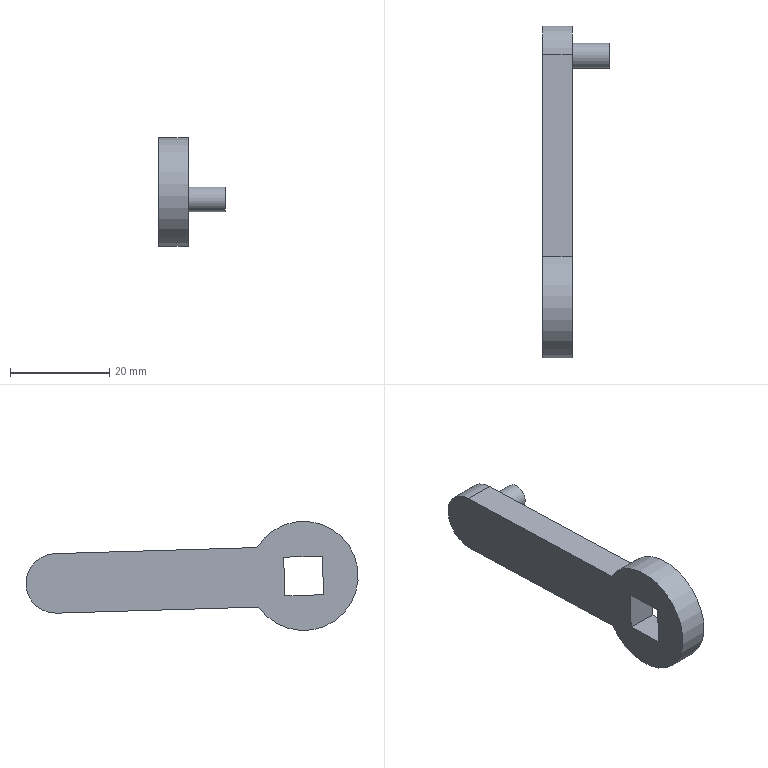Component | NX | ROCKER_CONNECTING_ROD | 1 solid | 12 faces | box 13.5 x 66.98 x 22 mm | volume 5252 mm3 | plane 9 | cylinder 3 | commonest cylinder face diameters 12 x1 22 x1 5 x1
STEP:
#1=CARTESIAN_POINT('',(0.,0.,0.));
#2=DIRECTION('',(0.,0.,1.));
#3=DIRECTION('',(1.,0.,0.));
#4=AXIS2_PLACEMENT_3D('',#1,#2,#3);
#5=CARTESIAN_POINT('',(35.,76.197,-15.982));
#6=VERTEX_POINT('',#5);
#7=CARTESIAN_POINT('',(35.,83.993,-16.221));
#8=VERTEX_POINT('',#7);
#9=CARTESIAN_POINT('',(35.,80.095,-16.101));
#10=DIRECTION('',(0.,0.9995,-0.03066));
#11=VECTOR('',#10,1.);
#12=LINE('',#9,#11);
#13=CARTESIAN_POINT('',(35.,129.953,-21.501));
#14=DIRECTION('',(1.,0.,0.));
#15=DIRECTION('',(0.,0.9995,-0.03004));
#16=AXIS2_PLACEMENT_3D('',#13,#14,#15);
#17=PLANE('',#16);
#18=CARTESIAN_POINT('',(-49.998,3.9));
#19=DIRECTION('',(1.,-0.000613));
#20=VECTOR('',#19,1.);
#21=LINE('',#18,#20);
#22=(GEOMETRIC_REPRESENTATION_CONTEXT(2)PARAMETRIC_REPRESENTATION_CONTEXT()REPRESENTATION_CONTEXT('',''));
#23=DEFINITIONAL_REPRESENTATION('',(#21),#22);
#24=PCURVE('',#17,#23);
#25=CARTESIAN_POINT('',(41.,84.093,-16.224));
#26=DIRECTION('',(0.,-0.03066,-0.9995));
#27=DIRECTION('',(0.,0.9995,-0.03066));
#28=AXIS2_PLACEMENT_3D('',#25,#26,#27);
#29=PLANE('',#28);
#30=CARTESIAN_POINT('',(-4.,-6.));
#31=DIRECTION('',(1.,0.));
#32=VECTOR('',#31,1.);
#33=LINE('',#30,#32);
#34=(GEOMETRIC_REPRESENTATION_CONTEXT(2)PARAMETRIC_REPRESENTATION_CONTEXT()REPRESENTATION_CONTEXT('',''));
#35=DEFINITIONAL_REPRESENTATION('',(#33),#34);
#36=PCURVE('',#29,#35);
#37=SURFACE_CURVE('',#12,(#24,#36),.PCURVE_S1.);
#38=EDGE_CURVE('',#6,#8,#37,.T.);
#39=ORIENTED_EDGE('',*,*,#38,.F.);
#40=CARTESIAN_POINT('',(35.,75.958,-23.778));
#41=VERTEX_POINT('',#40);
#42=CARTESIAN_POINT('',(35.,76.077,-19.88));
#43=DIRECTION('',(0.,0.03066,0.9995));
#44=VECTOR('',#43,1.);
#45=LINE('',#42,#44);
#46=CARTESIAN_POINT('',(-53.9,0.002391));
#47=DIRECTION('',(0.000613,1.));
#48=VECTOR('',#47,1.);
#49=LINE('',#46,#48);
#50=(GEOMETRIC_REPRESENTATION_CONTEXT(2)PARAMETRIC_REPRESENTATION_CONTEXT()REPRESENTATION_CONTEXT('',''));
#51=DEFINITIONAL_REPRESENTATION('',(#49),#50);
#52=PCURVE('',#17,#51);
#53=CARTESIAN_POINT('',(41.,76.2,-15.882));
#54=DIRECTION('',(0.,0.9995,-0.03066));
#55=DIRECTION('',(-1.,0.,0.));
#56=AXIS2_PLACEMENT_3D('',#53,#54,#55);
#57=PLANE('',#56);
#58=CARTESIAN_POINT('',(6.,-4.));
#59=DIRECTION('',(0.,1.));
#60=VECTOR('',#59,1.);
#61=LINE('',#58,#60);
#62=(GEOMETRIC_REPRESENTATION_CONTEXT(2)PARAMETRIC_REPRESENTATION_CONTEXT()REPRESENTATION_CONTEXT('',''));
#63=DEFINITIONAL_REPRESENTATION('',(#61),#62);
#64=PCURVE('',#57,#63);
#65=SURFACE_CURVE('',#45,(#52,#64),.PCURVE_S1.);
#66=EDGE_CURVE('',#41,#6,#65,.T.);
#67=ORIENTED_EDGE('',*,*,#66,.F.);
#68=CARTESIAN_POINT('',(35.,83.754,-24.017));
#69=VERTEX_POINT('',#68);
#70=CARTESIAN_POINT('',(35.,79.856,-23.897));
#71=DIRECTION('',(0.,-0.9995,0.03066));
#72=VECTOR('',#71,1.);
#73=LINE('',#70,#72);
#74=CARTESIAN_POINT('',(-50.002,-3.9));
#75=DIRECTION('',(-1.,0.000613));
#76=VECTOR('',#75,1.);
#77=LINE('',#74,#76);
#78=(GEOMETRIC_REPRESENTATION_CONTEXT(2)PARAMETRIC_REPRESENTATION_CONTEXT()REPRESENTATION_CONTEXT('',''));
#79=DEFINITIONAL_REPRESENTATION('',(#77),#78);
#80=PCURVE('',#17,#79);
#81=CARTESIAN_POINT('',(41.,75.858,-23.775));
#82=DIRECTION('',(0.,0.03066,0.9995));
#83=DIRECTION('',(0.,-0.9995,0.03066));
#84=AXIS2_PLACEMENT_3D('',#81,#82,#83);
#85=PLANE('',#84);
#86=CARTESIAN_POINT('',(-4.,-6.));
#87=DIRECTION('',(1.,0.));
#88=VECTOR('',#87,1.);
#89=LINE('',#86,#88);
#90=(GEOMETRIC_REPRESENTATION_CONTEXT(2)PARAMETRIC_REPRESENTATION_CONTEXT()REPRESENTATION_CONTEXT('',''));
#91=DEFINITIONAL_REPRESENTATION('',(#89),#90);
#92=PCURVE('',#85,#91);
#93=SURFACE_CURVE('',#73,(#80,#92),.PCURVE_S1.);
#94=EDGE_CURVE('',#69,#41,#93,.T.);
#95=ORIENTED_EDGE('',*,*,#94,.F.);
#96=CARTESIAN_POINT('',(35.,83.873,-20.119));
#97=DIRECTION('',(0.,-0.03066,-0.9995));
#98=VECTOR('',#97,1.);
#99=LINE('',#96,#98);
#100=CARTESIAN_POINT('',(-46.1,-0.002391));
#101=DIRECTION('',(-0.000613,-1.));
#102=VECTOR('',#101,1.);
#103=LINE('',#100,#102);
#104=(GEOMETRIC_REPRESENTATION_CONTEXT(2)PARAMETRIC_REPRESENTATION_CONTEXT()REPRESENTATION_CONTEXT('',''));
#105=DEFINITIONAL_REPRESENTATION('',(#103),#104);
#106=PCURVE('',#17,#105);
#107=CARTESIAN_POINT('',(41.,83.751,-24.117));
#108=DIRECTION('',(0.,-0.9995,0.03066));
#109=DIRECTION('',(0.,-0.03066,-0.9995));
#110=AXIS2_PLACEMENT_3D('',#107,#108,#109);
#111=PLANE('',#110);
#112=CARTESIAN_POINT('',(-4.,-6.));
#113=DIRECTION('',(1.,0.));
#114=VECTOR('',#113,1.);
#115=LINE('',#112,#114);
#116=(GEOMETRIC_REPRESENTATION_CONTEXT(2)PARAMETRIC_REPRESENTATION_CONTEXT()REPRESENTATION_CONTEXT('',''));
#117=DEFINITIONAL_REPRESENTATION('',(#115),#116);
#118=PCURVE('',#111,#117);
#119=SURFACE_CURVE('',#99,(#106,#118),.PCURVE_S1.);
#120=EDGE_CURVE('',#8,#69,#119,.T.);
#121=ORIENTED_EDGE('',*,*,#120,.F.);
#122=EDGE_LOOP('',(#39,#67,#95,#121));
#123=FACE_BOUND('',#122,.T.);
#124=CARTESIAN_POINT('',(35.,129.772,-27.499));
#125=VERTEX_POINT('',#124);
#126=CARTESIAN_POINT('',(35.,130.133,-15.504));
#127=VERTEX_POINT('',#126);
#128=CARTESIAN_POINT('',(35.,129.953,-21.501));
#129=DIRECTION('',(1.,0.,0.));
#130=DIRECTION('',(0.,-0.03004,-0.9995));
#131=AXIS2_PLACEMENT_3D('',#128,#129,#130);
#132=CIRCLE('',#131,6.);
#133=CARTESIAN_POINT('',(0.,0.));
#134=DIRECTION('',(-0.,-1.));
#135=AXIS2_PLACEMENT_2D('',#133,#134);
#136=CIRCLE('',#135,6.);
#137=(GEOMETRIC_REPRESENTATION_CONTEXT(2)PARAMETRIC_REPRESENTATION_CONTEXT()REPRESENTATION_CONTEXT('',''));
#138=DEFINITIONAL_REPRESENTATION('',(#136),#137);
#139=PCURVE('',#17,#138);
#140=CARTESIAN_POINT('',(35.,129.953,-21.501));
#141=DIRECTION('',(1.,0.,0.));
#142=DIRECTION('',(0.,0.9995,-0.03004));
#143=AXIS2_PLACEMENT_3D('',#140,#141,#142);
#144=CYLINDRICAL_SURFACE('',#143,6.);
#145=CARTESIAN_POINT('',(-1.571,0.));
#146=DIRECTION('',(1.,0.));
#147=VECTOR('',#146,1.);
#148=LINE('',#145,#147);
#149=(GEOMETRIC_REPRESENTATION_CONTEXT(2)PARAMETRIC_REPRESENTATION_CONTEXT()REPRESENTATION_CONTEXT('',''));
#150=DEFINITIONAL_REPRESENTATION('',(#148),#149);
#151=PCURVE('',#144,#150);
#152=SURFACE_CURVE('',#132,(#139,#151),.PCURVE_S1.);
#153=EDGE_CURVE('',#125,#127,#152,.T.);
#154=ORIENTED_EDGE('',*,*,#153,.F.);
#155=CARTESIAN_POINT('',(35.,89.01,-26.274));
#156=VERTEX_POINT('',#155);
#157=CARTESIAN_POINT('',(35.,89.01,-26.274));
#158=DIRECTION('',(0.,0.9995,-0.03004));
#159=VECTOR('',#158,1.);
#160=LINE('',#157,#159);
#161=CARTESIAN_POINT('',(-40.78,-6.));
#162=DIRECTION('',(1.,-0.));
#163=VECTOR('',#162,1.);
#164=LINE('',#161,#163);
#165=(GEOMETRIC_REPRESENTATION_CONTEXT(2)PARAMETRIC_REPRESENTATION_CONTEXT()REPRESENTATION_CONTEXT('',''));
#166=DEFINITIONAL_REPRESENTATION('',(#164),#165);
#167=PCURVE('',#17,#166);
#168=CARTESIAN_POINT('',(35.,89.01,-26.274));
#169=DIRECTION('',(0.,-0.03004,-0.9995));
#170=DIRECTION('',(0.,0.9995,-0.03004));
#171=AXIS2_PLACEMENT_3D('',#168,#169,#170);
#172=PLANE('',#171);
#173=CARTESIAN_POINT('',(0.,0.));
#174=DIRECTION('',(1.,0.));
#175=VECTOR('',#174,1.);
#176=LINE('',#173,#175);
#177=(GEOMETRIC_REPRESENTATION_CONTEXT(2)PARAMETRIC_REPRESENTATION_CONTEXT()REPRESENTATION_CONTEXT('',''));
#178=DEFINITIONAL_REPRESENTATION('',(#176),#177);
#179=PCURVE('',#172,#178);
#180=SURFACE_CURVE('',#160,(#167,#179),.PCURVE_S1.);
#181=EDGE_CURVE('',#156,#125,#180,.T.);
#182=ORIENTED_EDGE('',*,*,#181,.F.);
#183=CARTESIAN_POINT('',(35.,89.371,-14.279));
#184=VERTEX_POINT('',#183);
#185=CARTESIAN_POINT('',(35.,79.975,-19.999));
#186=DIRECTION('',(1.,0.,0.));
#187=DIRECTION('',(0.,-0.03004,-0.9995));
#188=AXIS2_PLACEMENT_3D('',#185,#186,#187);
#189=CIRCLE('',#188,11.);
#190=CARTESIAN_POINT('',(-50.,0.));
#191=DIRECTION('',(0.,-1.));
#192=AXIS2_PLACEMENT_2D('',#190,#191);
#193=CIRCLE('',#192,11.);
#194=(GEOMETRIC_REPRESENTATION_CONTEXT(2)PARAMETRIC_REPRESENTATION_CONTEXT()REPRESENTATION_CONTEXT('',''));
#195=DEFINITIONAL_REPRESENTATION('',(#193),#194);
#196=PCURVE('',#17,#195);
#197=CARTESIAN_POINT('',(35.,79.975,-19.999));
#198=DIRECTION('',(1.,0.,0.));
#199=DIRECTION('',(0.,0.9995,-0.03004));
#200=AXIS2_PLACEMENT_3D('',#197,#198,#199);
#201=CYLINDRICAL_SURFACE('',#200,11.);
#202=CARTESIAN_POINT('',(-1.571,0.));
#203=DIRECTION('',(1.,0.));
#204=VECTOR('',#203,1.);
#205=LINE('',#202,#204);
#206=(GEOMETRIC_REPRESENTATION_CONTEXT(2)PARAMETRIC_REPRESENTATION_CONTEXT()REPRESENTATION_CONTEXT('',''));
#207=DEFINITIONAL_REPRESENTATION('',(#205),#206);
#208=PCURVE('',#201,#207);
#209=SURFACE_CURVE('',#189,(#196,#208),.PCURVE_S1.);
#210=EDGE_CURVE('',#184,#156,#209,.T.);
#211=ORIENTED_EDGE('',*,*,#210,.F.);
#212=CARTESIAN_POINT('',(35.,130.133,-15.504));
#213=DIRECTION('',(0.,-0.9995,0.03004));
#214=VECTOR('',#213,1.);
#215=LINE('',#212,#214);
#216=CARTESIAN_POINT('',(-0.,6.));
#217=DIRECTION('',(-1.,0.));
#218=VECTOR('',#217,1.);
#219=LINE('',#216,#218);
#220=(GEOMETRIC_REPRESENTATION_CONTEXT(2)PARAMETRIC_REPRESENTATION_CONTEXT()REPRESENTATION_CONTEXT('',''));
#221=DEFINITIONAL_REPRESENTATION('',(#219),#220);
#222=PCURVE('',#17,#221);
#223=CARTESIAN_POINT('',(35.,130.133,-15.504));
#224=DIRECTION('',(0.,0.03004,0.9995));
#225=DIRECTION('',(0.,-0.9995,0.03004));
#226=AXIS2_PLACEMENT_3D('',#223,#224,#225);
#227=PLANE('',#226);
#228=CARTESIAN_POINT('',(0.,0.));
#229=DIRECTION('',(1.,0.));
#230=VECTOR('',#229,1.);
#231=LINE('',#228,#230);
#232=(GEOMETRIC_REPRESENTATION_CONTEXT(2)PARAMETRIC_REPRESENTATION_CONTEXT()REPRESENTATION_CONTEXT('',''));
#233=DEFINITIONAL_REPRESENTATION('',(#231),#232);
#234=PCURVE('',#227,#233);
#235=SURFACE_CURVE('',#215,(#222,#234),.PCURVE_S1.);
#236=EDGE_CURVE('',#127,#184,#235,.T.);
#237=ORIENTED_EDGE('',*,*,#236,.F.);
#238=EDGE_LOOP('',(#154,#182,#211,#237));
#239=FACE_BOUND('',#238,.T.);
#240=ADVANCED_FACE('',(#123,#239),#17,.F.);
#241=CARTESIAN_POINT('',(41.,129.878,-24.));
#242=VERTEX_POINT('',#241);
#243=CARTESIAN_POINT('',(41.,129.953,-21.501));
#244=DIRECTION('',(-1.,0.,0.));
#245=DIRECTION('',(0.,-0.03004,-0.9995));
#246=AXIS2_PLACEMENT_3D('',#243,#244,#245);
#247=CIRCLE('',#246,2.5);
#248=CARTESIAN_POINT('',(41.,129.953,-21.501));
#249=DIRECTION('',(1.,0.,0.));
#250=DIRECTION('',(0.,0.9995,-0.03004));
#251=AXIS2_PLACEMENT_3D('',#248,#249,#250);
#252=PLANE('',#251);
#253=CARTESIAN_POINT('',(0.,-2.5));
#254=CARTESIAN_POINT('',(-4.33,-2.5));
#255=CARTESIAN_POINT('',(-2.165,1.25));
#256=CARTESIAN_POINT('',(-0.,5.));
#257=CARTESIAN_POINT('',(2.165,1.25));
#258=CARTESIAN_POINT('',(4.33,-2.5));
#259=CARTESIAN_POINT('',(0.,-2.5));
#260=(BOUNDED_CURVE()B_SPLINE_CURVE(2,(#253,#254,#255,#256,#257,#258,#259),.UNSPECIFIED.,.T.,.F.)B_SPLINE_CURVE_WITH_KNOTS((1,2,2,2,2,1),(-2.094,0.,2.094,4.189,6.283,8.378),.UNSPECIFIED.)CURVE()GEOMETRIC_REPRESENTATION_ITEM()RATIONAL_B_SPLINE_CURVE((1.,0.5,1.,0.5,1.,0.5,1.))REPRESENTATION_ITEM(''));
#261=(GEOMETRIC_REPRESENTATION_CONTEXT(2)PARAMETRIC_REPRESENTATION_CONTEXT()REPRESENTATION_CONTEXT('',''));
#262=DEFINITIONAL_REPRESENTATION('',(#260),#261);
#263=PCURVE('',#252,#262);
#264=CARTESIAN_POINT('',(48.5,129.953,-21.501));
#265=DIRECTION('',(-1.,0.,0.));
#266=DIRECTION('',(0.,-0.9995,0.03004));
#267=AXIS2_PLACEMENT_3D('',#264,#265,#266);
#268=CYLINDRICAL_SURFACE('',#267,2.5);
#269=CARTESIAN_POINT('',(4.712,7.5));
#270=DIRECTION('',(1.,0.));
#271=VECTOR('',#270,1.);
#272=LINE('',#269,#271);
#273=(GEOMETRIC_REPRESENTATION_CONTEXT(2)PARAMETRIC_REPRESENTATION_CONTEXT()REPRESENTATION_CONTEXT('',''));
#274=DEFINITIONAL_REPRESENTATION('',(#272),#273);
#275=PCURVE('',#268,#274);
#276=SURFACE_CURVE('',#247,(#263,#275),.PCURVE_S1.);
#277=EDGE_CURVE('',#242,#242,#276,.T.);
#278=ORIENTED_EDGE('',*,*,#277,.T.);
#279=EDGE_LOOP('',(#278));
#280=FACE_BOUND('',#279,.T.);
#281=CARTESIAN_POINT('',(41.,129.772,-27.499));
#282=VERTEX_POINT('',#281);
#283=CARTESIAN_POINT('',(41.,130.133,-15.504));
#284=VERTEX_POINT('',#283);
#285=CARTESIAN_POINT('',(41.,129.953,-21.501));
#286=DIRECTION('',(1.,0.,0.));
#287=DIRECTION('',(0.,-0.03004,-0.9995));
#288=AXIS2_PLACEMENT_3D('',#285,#286,#287);
#289=CIRCLE('',#288,6.);
#290=CARTESIAN_POINT('',(0.,0.));
#291=DIRECTION('',(-0.,-1.));
#292=AXIS2_PLACEMENT_2D('',#290,#291);
#293=CIRCLE('',#292,6.);
#294=(GEOMETRIC_REPRESENTATION_CONTEXT(2)PARAMETRIC_REPRESENTATION_CONTEXT()REPRESENTATION_CONTEXT('',''));
#295=DEFINITIONAL_REPRESENTATION('',(#293),#294);
#296=PCURVE('',#252,#295);
#297=CARTESIAN_POINT('',(-1.571,6.));
#298=DIRECTION('',(1.,0.));
#299=VECTOR('',#298,1.);
#300=LINE('',#297,#299);
#301=(GEOMETRIC_REPRESENTATION_CONTEXT(2)PARAMETRIC_REPRESENTATION_CONTEXT()REPRESENTATION_CONTEXT('',''));
#302=DEFINITIONAL_REPRESENTATION('',(#300),#301);
#303=PCURVE('',#144,#302);
#304=SURFACE_CURVE('',#289,(#296,#303),.PCURVE_S1.);
#305=EDGE_CURVE('',#282,#284,#304,.T.);
#306=ORIENTED_EDGE('',*,*,#305,.T.);
#307=CARTESIAN_POINT('',(41.,89.371,-14.279));
#308=VERTEX_POINT('',#307);
#309=CARTESIAN_POINT('',(41.,130.133,-15.504));
#310=DIRECTION('',(0.,-0.9995,0.03004));
#311=VECTOR('',#310,1.);
#312=LINE('',#309,#311);
#313=CARTESIAN_POINT('',(-0.,6.));
#314=DIRECTION('',(-1.,0.));
#315=VECTOR('',#314,1.);
#316=LINE('',#313,#315);
#317=(GEOMETRIC_REPRESENTATION_CONTEXT(2)PARAMETRIC_REPRESENTATION_CONTEXT()REPRESENTATION_CONTEXT('',''));
#318=DEFINITIONAL_REPRESENTATION('',(#316),#317);
#319=PCURVE('',#252,#318);
#320=CARTESIAN_POINT('',(0.,6.));
#321=DIRECTION('',(1.,0.));
#322=VECTOR('',#321,1.);
#323=LINE('',#320,#322);
#324=(GEOMETRIC_REPRESENTATION_CONTEXT(2)PARAMETRIC_REPRESENTATION_CONTEXT()REPRESENTATION_CONTEXT('',''));
#325=DEFINITIONAL_REPRESENTATION('',(#323),#324);
#326=PCURVE('',#227,#325);
#327=SURFACE_CURVE('',#312,(#319,#326),.PCURVE_S1.);
#328=EDGE_CURVE('',#284,#308,#327,.T.);
#329=ORIENTED_EDGE('',*,*,#328,.T.);
#330=CARTESIAN_POINT('',(41.,89.01,-26.274));
#331=VERTEX_POINT('',#330);
#332=CARTESIAN_POINT('',(41.,79.975,-19.999));
#333=DIRECTION('',(1.,0.,0.));
#334=DIRECTION('',(0.,-0.03004,-0.9995));
#335=AXIS2_PLACEMENT_3D('',#332,#333,#334);
#336=CIRCLE('',#335,11.);
#337=CARTESIAN_POINT('',(-50.,0.));
#338=DIRECTION('',(0.,-1.));
#339=AXIS2_PLACEMENT_2D('',#337,#338);
#340=CIRCLE('',#339,11.);
#341=(GEOMETRIC_REPRESENTATION_CONTEXT(2)PARAMETRIC_REPRESENTATION_CONTEXT()REPRESENTATION_CONTEXT('',''));
#342=DEFINITIONAL_REPRESENTATION('',(#340),#341);
#343=PCURVE('',#252,#342);
#344=CARTESIAN_POINT('',(-1.571,6.));
#345=DIRECTION('',(1.,0.));
#346=VECTOR('',#345,1.);
#347=LINE('',#344,#346);
#348=(GEOMETRIC_REPRESENTATION_CONTEXT(2)PARAMETRIC_REPRESENTATION_CONTEXT()REPRESENTATION_CONTEXT('',''));
#349=DEFINITIONAL_REPRESENTATION('',(#347),#348);
#350=PCURVE('',#201,#349);
#351=SURFACE_CURVE('',#336,(#343,#350),.PCURVE_S1.);
#352=EDGE_CURVE('',#308,#331,#351,.T.);
#353=ORIENTED_EDGE('',*,*,#352,.T.);
#354=CARTESIAN_POINT('',(41.,89.01,-26.274));
#355=DIRECTION('',(0.,0.9995,-0.03004));
#356=VECTOR('',#355,1.);
#357=LINE('',#354,#356);
#358=CARTESIAN_POINT('',(-40.78,-6.));
#359=DIRECTION('',(1.,-0.));
#360=VECTOR('',#359,1.);
#361=LINE('',#358,#360);
#362=(GEOMETRIC_REPRESENTATION_CONTEXT(2)PARAMETRIC_REPRESENTATION_CONTEXT()REPRESENTATION_CONTEXT('',''));
#363=DEFINITIONAL_REPRESENTATION('',(#361),#362);
#364=PCURVE('',#252,#363);
#365=CARTESIAN_POINT('',(0.,6.));
#366=DIRECTION('',(1.,0.));
#367=VECTOR('',#366,1.);
#368=LINE('',#365,#367);
#369=(GEOMETRIC_REPRESENTATION_CONTEXT(2)PARAMETRIC_REPRESENTATION_CONTEXT()REPRESENTATION_CONTEXT('',''));
#370=DEFINITIONAL_REPRESENTATION('',(#368),#369);
#371=PCURVE('',#172,#370);
#372=SURFACE_CURVE('',#357,(#364,#371),.PCURVE_S1.);
#373=EDGE_CURVE('',#331,#282,#372,.T.);
#374=ORIENTED_EDGE('',*,*,#373,.T.);
#375=EDGE_LOOP('',(#306,#329,#353,#374));
#376=FACE_BOUND('',#375,.T.);
#377=CARTESIAN_POINT('',(41.,76.197,-15.982));
#378=VERTEX_POINT('',#377);
#379=CARTESIAN_POINT('',(41.,75.958,-23.778));
#380=VERTEX_POINT('',#379);
#381=CARTESIAN_POINT('',(41.,76.2,-15.882));
#382=DIRECTION('',(0.,-0.03066,-0.9995));
#383=VECTOR('',#382,1.);
#384=LINE('',#381,#383);
#385=CARTESIAN_POINT('',(-53.898,4.002));
#386=DIRECTION('',(-0.000613,-1.));
#387=VECTOR('',#386,1.);
#388=LINE('',#385,#387);
#389=(GEOMETRIC_REPRESENTATION_CONTEXT(2)PARAMETRIC_REPRESENTATION_CONTEXT()REPRESENTATION_CONTEXT('',''));
#390=DEFINITIONAL_REPRESENTATION('',(#388),#389);
#391=PCURVE('',#252,#390);
#392=CARTESIAN_POINT('',(0.,0.));
#393=DIRECTION('',(0.,-1.));
#394=VECTOR('',#393,1.);
#395=LINE('',#392,#394);
#396=(GEOMETRIC_REPRESENTATION_CONTEXT(2)PARAMETRIC_REPRESENTATION_CONTEXT()REPRESENTATION_CONTEXT('',''));
#397=DEFINITIONAL_REPRESENTATION('',(#395),#396);
#398=PCURVE('',#57,#397);
#399=SURFACE_CURVE('',#384,(#391,#398),.PCURVE_S1.);
#400=EDGE_CURVE('',#378,#380,#399,.T.);
#401=ORIENTED_EDGE('',*,*,#400,.F.);
#402=CARTESIAN_POINT('',(41.,83.993,-16.221));
#403=VERTEX_POINT('',#402);
#404=CARTESIAN_POINT('',(41.,84.093,-16.224));
#405=DIRECTION('',(0.,-0.9995,0.03066));
#406=VECTOR('',#405,1.);
#407=LINE('',#404,#406);
#408=CARTESIAN_POINT('',(-45.998,3.898));
#409=DIRECTION('',(-1.,0.000613));
#410=VECTOR('',#409,1.);
#411=LINE('',#408,#410);
#412=(GEOMETRIC_REPRESENTATION_CONTEXT(2)PARAMETRIC_REPRESENTATION_CONTEXT()REPRESENTATION_CONTEXT('',''));
#413=DEFINITIONAL_REPRESENTATION('',(#411),#412);
#414=PCURVE('',#252,#413);
#415=CARTESIAN_POINT('',(0.,0.));
#416=DIRECTION('',(-1.,0.));
#417=VECTOR('',#416,1.);
#418=LINE('',#415,#417);
#419=(GEOMETRIC_REPRESENTATION_CONTEXT(2)PARAMETRIC_REPRESENTATION_CONTEXT()REPRESENTATION_CONTEXT('',''));
#420=DEFINITIONAL_REPRESENTATION('',(#418),#419);
#421=PCURVE('',#29,#420);
#422=SURFACE_CURVE('',#407,(#414,#421),.PCURVE_S1.);
#423=EDGE_CURVE('',#403,#378,#422,.T.);
#424=ORIENTED_EDGE('',*,*,#423,.F.);
#425=CARTESIAN_POINT('',(41.,83.754,-24.017));
#426=VERTEX_POINT('',#425);
#427=CARTESIAN_POINT('',(41.,83.751,-24.117));
#428=DIRECTION('',(0.,0.03066,0.9995));
#429=VECTOR('',#428,1.);
#430=LINE('',#427,#429);
#431=CARTESIAN_POINT('',(-46.102,-4.002));
#432=DIRECTION('',(0.000613,1.));
#433=VECTOR('',#432,1.);
#434=LINE('',#431,#433);
#435=(GEOMETRIC_REPRESENTATION_CONTEXT(2)PARAMETRIC_REPRESENTATION_CONTEXT()REPRESENTATION_CONTEXT('',''));
#436=DEFINITIONAL_REPRESENTATION('',(#434),#435);
#437=PCURVE('',#252,#436);
#438=CARTESIAN_POINT('',(0.,0.));
#439=DIRECTION('',(-1.,0.));
#440=VECTOR('',#439,1.);
#441=LINE('',#438,#440);
#442=(GEOMETRIC_REPRESENTATION_CONTEXT(2)PARAMETRIC_REPRESENTATION_CONTEXT()REPRESENTATION_CONTEXT('',''));
#443=DEFINITIONAL_REPRESENTATION('',(#441),#442);
#444=PCURVE('',#111,#443);
#445=SURFACE_CURVE('',#430,(#437,#444),.PCURVE_S1.);
#446=EDGE_CURVE('',#426,#403,#445,.T.);
#447=ORIENTED_EDGE('',*,*,#446,.F.);
#448=CARTESIAN_POINT('',(41.,75.858,-23.775));
#449=DIRECTION('',(0.,0.9995,-0.03066));
#450=VECTOR('',#449,1.);
#451=LINE('',#448,#450);
#452=CARTESIAN_POINT('',(-54.002,-3.898));
#453=DIRECTION('',(1.,-0.000613));
#454=VECTOR('',#453,1.);
#455=LINE('',#452,#454);
#456=(GEOMETRIC_REPRESENTATION_CONTEXT(2)PARAMETRIC_REPRESENTATION_CONTEXT()REPRESENTATION_CONTEXT('',''));
#457=DEFINITIONAL_REPRESENTATION('',(#455),#456);
#458=PCURVE('',#252,#457);
#459=CARTESIAN_POINT('',(0.,0.));
#460=DIRECTION('',(-1.,0.));
#461=VECTOR('',#460,1.);
#462=LINE('',#459,#461);
#463=(GEOMETRIC_REPRESENTATION_CONTEXT(2)PARAMETRIC_REPRESENTATION_CONTEXT()REPRESENTATION_CONTEXT('',''));
#464=DEFINITIONAL_REPRESENTATION('',(#462),#463);
#465=PCURVE('',#85,#464);
#466=SURFACE_CURVE('',#451,(#458,#465),.PCURVE_S1.);
#467=EDGE_CURVE('',#380,#426,#466,.T.);
#468=ORIENTED_EDGE('',*,*,#467,.F.);
#469=EDGE_LOOP('',(#401,#424,#447,#468));
#470=FACE_BOUND('',#469,.T.);
#471=ADVANCED_FACE('',(#280,#376,#470),#252,.T.);
#472=ORIENTED_EDGE('',*,*,#305,.F.);
#473=CARTESIAN_POINT('',(35.,129.772,-27.499));
#474=DIRECTION('',(1.,0.,0.));
#475=VECTOR('',#474,1.);
#476=LINE('',#473,#475);
#477=CARTESIAN_POINT('',(-1.571,0.));
#478=DIRECTION('',(0.,1.));
#479=VECTOR('',#478,1.);
#480=LINE('',#477,#479);
#481=(GEOMETRIC_REPRESENTATION_CONTEXT(2)PARAMETRIC_REPRESENTATION_CONTEXT()REPRESENTATION_CONTEXT('',''));
#482=DEFINITIONAL_REPRESENTATION('',(#480),#481);
#483=PCURVE('',#144,#482);
#484=CARTESIAN_POINT('',(40.78,0.));
#485=DIRECTION('',(0.,1.));
#486=VECTOR('',#485,1.);
#487=LINE('',#484,#486);
#488=(GEOMETRIC_REPRESENTATION_CONTEXT(2)PARAMETRIC_REPRESENTATION_CONTEXT()REPRESENTATION_CONTEXT('',''));
#489=DEFINITIONAL_REPRESENTATION('',(#487),#488);
#490=PCURVE('',#172,#489);
#491=SURFACE_CURVE('',#476,(#483,#490),.PCURVE_S1.);
#492=EDGE_CURVE('',#125,#282,#491,.T.);
#493=ORIENTED_EDGE('',*,*,#492,.F.);
#494=ORIENTED_EDGE('',*,*,#153,.T.);
#495=CARTESIAN_POINT('',(35.,130.133,-15.504));
#496=DIRECTION('',(1.,0.,0.));
#497=VECTOR('',#496,1.);
#498=LINE('',#495,#497);
#499=CARTESIAN_POINT('',(1.571,0.));
#500=DIRECTION('',(0.,1.));
#501=VECTOR('',#500,1.);
#502=LINE('',#499,#501);
#503=(GEOMETRIC_REPRESENTATION_CONTEXT(2)PARAMETRIC_REPRESENTATION_CONTEXT()REPRESENTATION_CONTEXT('',''));
#504=DEFINITIONAL_REPRESENTATION('',(#502),#503);
#505=PCURVE('',#144,#504);
#506=CARTESIAN_POINT('',(0.,0.));
#507=DIRECTION('',(0.,1.));
#508=VECTOR('',#507,1.);
#509=LINE('',#506,#508);
#510=(GEOMETRIC_REPRESENTATION_CONTEXT(2)PARAMETRIC_REPRESENTATION_CONTEXT()REPRESENTATION_CONTEXT('',''));
#511=DEFINITIONAL_REPRESENTATION('',(#509),#510);
#512=PCURVE('',#227,#511);
#513=SURFACE_CURVE('',#498,(#505,#512),.PCURVE_S1.);
#514=EDGE_CURVE('',#127,#284,#513,.T.);
#515=ORIENTED_EDGE('',*,*,#514,.T.);
#516=EDGE_LOOP('',(#472,#493,#494,#515));
#517=FACE_BOUND('',#516,.T.);
#518=ADVANCED_FACE('',(#517),#144,.T.);
#519=ORIENTED_EDGE('',*,*,#328,.F.);
#520=ORIENTED_EDGE('',*,*,#514,.F.);
#521=ORIENTED_EDGE('',*,*,#236,.T.);
#522=CARTESIAN_POINT('',(35.,89.371,-14.279));
#523=DIRECTION('',(1.,0.,0.));
#524=VECTOR('',#523,1.);
#525=LINE('',#522,#524);
#526=CARTESIAN_POINT('',(40.78,0.));
#527=DIRECTION('',(0.,1.));
#528=VECTOR('',#527,1.);
#529=LINE('',#526,#528);
#530=(GEOMETRIC_REPRESENTATION_CONTEXT(2)PARAMETRIC_REPRESENTATION_CONTEXT()REPRESENTATION_CONTEXT('',''));
#531=DEFINITIONAL_REPRESENTATION('',(#529),#530);
#532=PCURVE('',#227,#531);
#533=CARTESIAN_POINT('',(0.5769,0.));
#534=DIRECTION('',(0.,1.));
#535=VECTOR('',#534,1.);
#536=LINE('',#533,#535);
#537=(GEOMETRIC_REPRESENTATION_CONTEXT(2)PARAMETRIC_REPRESENTATION_CONTEXT()REPRESENTATION_CONTEXT('',''));
#538=DEFINITIONAL_REPRESENTATION('',(#536),#537);
#539=PCURVE('',#201,#538);
#540=SURFACE_CURVE('',#525,(#532,#539),.PCURVE_S1.);
#541=EDGE_CURVE('',#184,#308,#540,.T.);
#542=ORIENTED_EDGE('',*,*,#541,.T.);
#543=EDGE_LOOP('',(#519,#520,#521,#542));
#544=FACE_BOUND('',#543,.T.);
#545=ADVANCED_FACE('',(#544),#227,.T.);
#546=ORIENTED_EDGE('',*,*,#352,.F.);
#547=ORIENTED_EDGE('',*,*,#541,.F.);
#548=ORIENTED_EDGE('',*,*,#210,.T.);
#549=CARTESIAN_POINT('',(35.,89.01,-26.274));
#550=DIRECTION('',(1.,0.,0.));
#551=VECTOR('',#550,1.);
#552=LINE('',#549,#551);
#553=CARTESIAN_POINT('',(5.706,0.));
#554=DIRECTION('',(0.,1.));
#555=VECTOR('',#554,1.);
#556=LINE('',#553,#555);
#557=(GEOMETRIC_REPRESENTATION_CONTEXT(2)PARAMETRIC_REPRESENTATION_CONTEXT()REPRESENTATION_CONTEXT('',''));
#558=DEFINITIONAL_REPRESENTATION('',(#556),#557);
#559=PCURVE('',#201,#558);
#560=CARTESIAN_POINT('',(-0.,0.));
#561=DIRECTION('',(0.,1.));
#562=VECTOR('',#561,1.);
#563=LINE('',#560,#562);
#564=(GEOMETRIC_REPRESENTATION_CONTEXT(2)PARAMETRIC_REPRESENTATION_CONTEXT()REPRESENTATION_CONTEXT('',''));
#565=DEFINITIONAL_REPRESENTATION('',(#563),#564);
#566=PCURVE('',#172,#565);
#567=SURFACE_CURVE('',#552,(#559,#566),.PCURVE_S1.);
#568=EDGE_CURVE('',#156,#331,#567,.T.);
#569=ORIENTED_EDGE('',*,*,#568,.T.);
#570=EDGE_LOOP('',(#546,#547,#548,#569));
#571=FACE_BOUND('',#570,.T.);
#572=ADVANCED_FACE('',(#571),#201,.T.);
#573=ORIENTED_EDGE('',*,*,#373,.F.);
#574=ORIENTED_EDGE('',*,*,#568,.F.);
#575=ORIENTED_EDGE('',*,*,#181,.T.);
#576=ORIENTED_EDGE('',*,*,#492,.T.);
#577=EDGE_LOOP('',(#573,#574,#575,#576));
#578=FACE_BOUND('',#577,.T.);
#579=ADVANCED_FACE('',(#578),#172,.T.);
#580=CARTESIAN_POINT('',(48.5,129.878,-24.));
#581=VERTEX_POINT('',#580);
#582=CARTESIAN_POINT('',(48.5,129.953,-21.501));
#583=DIRECTION('',(-1.,0.,0.));
#584=DIRECTION('',(0.,-0.03004,-0.9995));
#585=AXIS2_PLACEMENT_3D('',#582,#583,#584);
#586=CIRCLE('',#585,2.5);
#587=CARTESIAN_POINT('',(4.712,0.));
#588=DIRECTION('',(1.,0.));
#589=VECTOR('',#588,1.);
#590=LINE('',#587,#589);
#591=(GEOMETRIC_REPRESENTATION_CONTEXT(2)PARAMETRIC_REPRESENTATION_CONTEXT()REPRESENTATION_CONTEXT('',''));
#592=DEFINITIONAL_REPRESENTATION('',(#590),#591);
#593=PCURVE('',#268,#592);
#594=CARTESIAN_POINT('',(48.5,129.953,-21.501));
#595=DIRECTION('',(-1.,0.,0.));
#596=DIRECTION('',(0.,-0.9995,0.03004));
#597=AXIS2_PLACEMENT_3D('',#594,#595,#596);
#598=PLANE('',#597);
#599=CARTESIAN_POINT('',(0.,0.));
#600=DIRECTION('',(-0.,-1.));
#601=AXIS2_PLACEMENT_2D('',#599,#600);
#602=CIRCLE('',#601,2.5);
#603=(GEOMETRIC_REPRESENTATION_CONTEXT(2)PARAMETRIC_REPRESENTATION_CONTEXT()REPRESENTATION_CONTEXT('',''));
#604=DEFINITIONAL_REPRESENTATION('',(#602),#603);
#605=PCURVE('',#598,#604);
#606=SURFACE_CURVE('',#586,(#593,#605),.PCURVE_S1.);
#607=EDGE_CURVE('',#581,#581,#606,.T.);
#608=ORIENTED_EDGE('',*,*,#607,.T.);
#609=CARTESIAN_POINT('',(48.5,129.878,-24.));
#610=CARTESIAN_POINT('',(41.,129.878,-24.));
#611=B_SPLINE_CURVE_WITH_KNOTS('',1,(#609,#610),.UNSPECIFIED.,.F.,.F.,(2,2),(0.,7.5),.PIECEWISE_BEZIER_KNOTS.);
#612=CARTESIAN_POINT('',(10.996,0.));
#613=DIRECTION('',(0.,1.));
#614=VECTOR('',#613,1.);
#615=LINE('',#612,#614);
#616=(GEOMETRIC_REPRESENTATION_CONTEXT(2)PARAMETRIC_REPRESENTATION_CONTEXT()REPRESENTATION_CONTEXT('',''));
#617=DEFINITIONAL_REPRESENTATION('',(#615),#616);
#618=PCURVE('',#268,#617);
#619=CARTESIAN_POINT('',(4.712,0.));
#620=DIRECTION('',(0.,1.));
#621=VECTOR('',#620,1.);
#622=LINE('',#619,#621);
#623=(GEOMETRIC_REPRESENTATION_CONTEXT(2)PARAMETRIC_REPRESENTATION_CONTEXT()REPRESENTATION_CONTEXT('',''));
#624=DEFINITIONAL_REPRESENTATION('',(#622),#623);
#625=PCURVE('',#268,#624);
#626=SEAM_CURVE('',#611,(#618,#625),.PCURVE_S1.);
#627=EDGE_CURVE('',#581,#242,#626,.T.);
#628=ORIENTED_EDGE('',*,*,#627,.T.);
#629=ORIENTED_EDGE('',*,*,#277,.F.);
#630=ORIENTED_EDGE('',*,*,#627,.F.);
#631=EDGE_LOOP('',(#608,#628,#629,#630));
#632=FACE_BOUND('',#631,.T.);
#633=ADVANCED_FACE('',(#632),#268,.T.);
#634=ORIENTED_EDGE('',*,*,#607,.F.);
#635=EDGE_LOOP('',(#634));
#636=FACE_BOUND('',#635,.T.);
#637=ADVANCED_FACE('',(#636),#598,.F.);
#638=ORIENTED_EDGE('',*,*,#38,.T.);
#639=CARTESIAN_POINT('',(41.,83.993,-16.221));
#640=DIRECTION('',(1.,0.,0.));
#641=VECTOR('',#640,1.);
#642=LINE('',#639,#641);
#643=CARTESIAN_POINT('',(-0.1,0.));
#644=DIRECTION('',(0.,1.));
#645=VECTOR('',#644,1.);
#646=LINE('',#643,#645);
#647=(GEOMETRIC_REPRESENTATION_CONTEXT(2)PARAMETRIC_REPRESENTATION_CONTEXT()REPRESENTATION_CONTEXT('',''));
#648=DEFINITIONAL_REPRESENTATION('',(#646),#647);
#649=PCURVE('',#29,#648);
#650=CARTESIAN_POINT('',(-7.9,0.));
#651=DIRECTION('',(0.,1.));
#652=VECTOR('',#651,1.);
#653=LINE('',#650,#652);
#654=(GEOMETRIC_REPRESENTATION_CONTEXT(2)PARAMETRIC_REPRESENTATION_CONTEXT()REPRESENTATION_CONTEXT('',''));
#655=DEFINITIONAL_REPRESENTATION('',(#653),#654);
#656=PCURVE('',#111,#655);
#657=SURFACE_CURVE('',#642,(#649,#656),.PCURVE_S1.);
#658=EDGE_CURVE('',#8,#403,#657,.T.);
#659=ORIENTED_EDGE('',*,*,#658,.T.);
#660=ORIENTED_EDGE('',*,*,#423,.T.);
#661=CARTESIAN_POINT('',(41.,76.197,-15.982));
#662=DIRECTION('',(1.,0.,0.));
#663=VECTOR('',#662,1.);
#664=LINE('',#661,#663);
#665=CARTESIAN_POINT('',(-7.9,0.));
#666=DIRECTION('',(0.,1.));
#667=VECTOR('',#666,1.);
#668=LINE('',#665,#667);
#669=(GEOMETRIC_REPRESENTATION_CONTEXT(2)PARAMETRIC_REPRESENTATION_CONTEXT()REPRESENTATION_CONTEXT('',''));
#670=DEFINITIONAL_REPRESENTATION('',(#668),#669);
#671=PCURVE('',#29,#670);
#672=CARTESIAN_POINT('',(0.,-0.1));
#673=DIRECTION('',(-1.,0.));
#674=VECTOR('',#673,1.);
#675=LINE('',#672,#674);
#676=(GEOMETRIC_REPRESENTATION_CONTEXT(2)PARAMETRIC_REPRESENTATION_CONTEXT()REPRESENTATION_CONTEXT('',''));
#677=DEFINITIONAL_REPRESENTATION('',(#675),#676);
#678=PCURVE('',#57,#677);
#679=SURFACE_CURVE('',#664,(#671,#678),.PCURVE_S1.);
#680=EDGE_CURVE('',#6,#378,#679,.T.);
#681=ORIENTED_EDGE('',*,*,#680,.F.);
#682=EDGE_LOOP('',(#638,#659,#660,#681));
#683=FACE_BOUND('',#682,.T.);
#684=ADVANCED_FACE('',(#683),#29,.T.);
#685=ORIENTED_EDGE('',*,*,#66,.T.);
#686=ORIENTED_EDGE('',*,*,#680,.T.);
#687=ORIENTED_EDGE('',*,*,#400,.T.);
#688=CARTESIAN_POINT('',(41.,75.958,-23.778));
#689=DIRECTION('',(1.,0.,0.));
#690=VECTOR('',#689,1.);
#691=LINE('',#688,#690);
#692=CARTESIAN_POINT('',(0.,-7.9));
#693=DIRECTION('',(-1.,0.));
#694=VECTOR('',#693,1.);
#695=LINE('',#692,#694);
#696=(GEOMETRIC_REPRESENTATION_CONTEXT(2)PARAMETRIC_REPRESENTATION_CONTEXT()REPRESENTATION_CONTEXT('',''));
#697=DEFINITIONAL_REPRESENTATION('',(#695),#696);
#698=PCURVE('',#57,#697);
#699=CARTESIAN_POINT('',(-0.1,0.));
#700=DIRECTION('',(0.,1.));
#701=VECTOR('',#700,1.);
#702=LINE('',#699,#701);
#703=(GEOMETRIC_REPRESENTATION_CONTEXT(2)PARAMETRIC_REPRESENTATION_CONTEXT()REPRESENTATION_CONTEXT('',''));
#704=DEFINITIONAL_REPRESENTATION('',(#702),#703);
#705=PCURVE('',#85,#704);
#706=SURFACE_CURVE('',#691,(#698,#705),.PCURVE_S1.);
#707=EDGE_CURVE('',#41,#380,#706,.T.);
#708=ORIENTED_EDGE('',*,*,#707,.F.);
#709=EDGE_LOOP('',(#685,#686,#687,#708));
#710=FACE_BOUND('',#709,.T.);
#711=ADVANCED_FACE('',(#710),#57,.T.);
#712=ORIENTED_EDGE('',*,*,#94,.T.);
#713=ORIENTED_EDGE('',*,*,#707,.T.);
#714=ORIENTED_EDGE('',*,*,#467,.T.);
#715=CARTESIAN_POINT('',(41.,83.754,-24.017));
#716=DIRECTION('',(1.,0.,0.));
#717=VECTOR('',#716,1.);
#718=LINE('',#715,#717);
#719=CARTESIAN_POINT('',(-7.9,0.));
#720=DIRECTION('',(0.,1.));
#721=VECTOR('',#720,1.);
#722=LINE('',#719,#721);
#723=(GEOMETRIC_REPRESENTATION_CONTEXT(2)PARAMETRIC_REPRESENTATION_CONTEXT()REPRESENTATION_CONTEXT('',''));
#724=DEFINITIONAL_REPRESENTATION('',(#722),#723);
#725=PCURVE('',#85,#724);
#726=CARTESIAN_POINT('',(-0.1,0.));
#727=DIRECTION('',(0.,1.));
#728=VECTOR('',#727,1.);
#729=LINE('',#726,#728);
#730=(GEOMETRIC_REPRESENTATION_CONTEXT(2)PARAMETRIC_REPRESENTATION_CONTEXT()REPRESENTATION_CONTEXT('',''));
#731=DEFINITIONAL_REPRESENTATION('',(#729),#730);
#732=PCURVE('',#111,#731);
#733=SURFACE_CURVE('',#718,(#725,#732),.PCURVE_S1.);
#734=EDGE_CURVE('',#69,#426,#733,.T.);
#735=ORIENTED_EDGE('',*,*,#734,.F.);
#736=EDGE_LOOP('',(#712,#713,#714,#735));
#737=FACE_BOUND('',#736,.T.);
#738=ADVANCED_FACE('',(#737),#85,.T.);
#739=ORIENTED_EDGE('',*,*,#120,.T.);
#740=ORIENTED_EDGE('',*,*,#734,.T.);
#741=ORIENTED_EDGE('',*,*,#446,.T.);
#742=ORIENTED_EDGE('',*,*,#658,.F.);
#743=EDGE_LOOP('',(#739,#740,#741,#742));
#744=FACE_BOUND('',#743,.T.);
#745=ADVANCED_FACE('',(#744),#111,.T.);
#746=CLOSED_SHELL('',(#240,#471,#518,#545,#572,#579,#633,#637,#684,#711,#738,#745));
#747=MANIFOLD_SOLID_BREP('',#746);
#748=(LENGTH_UNIT()NAMED_UNIT(*)SI_UNIT(.MILLI.,.METRE.));
#749=UNCERTAINTY_MEASURE_WITH_UNIT(LENGTH_MEASURE(0.000001),#748,'','');
#750=(NAMED_UNIT(*)PLANE_ANGLE_UNIT()SI_UNIT($,.RADIAN.));
#751=(NAMED_UNIT(*)SI_UNIT($,.STERADIAN.)SOLID_ANGLE_UNIT());
#752=(GEOMETRIC_REPRESENTATION_CONTEXT(3)GLOBAL_UNCERTAINTY_ASSIGNED_CONTEXT((#749))GLOBAL_UNIT_ASSIGNED_CONTEXT((#748,#750,#751))REPRESENTATION_CONTEXT('',''));
#753=ADVANCED_BREP_SHAPE_REPRESENTATION('',(#4,#747),#752);